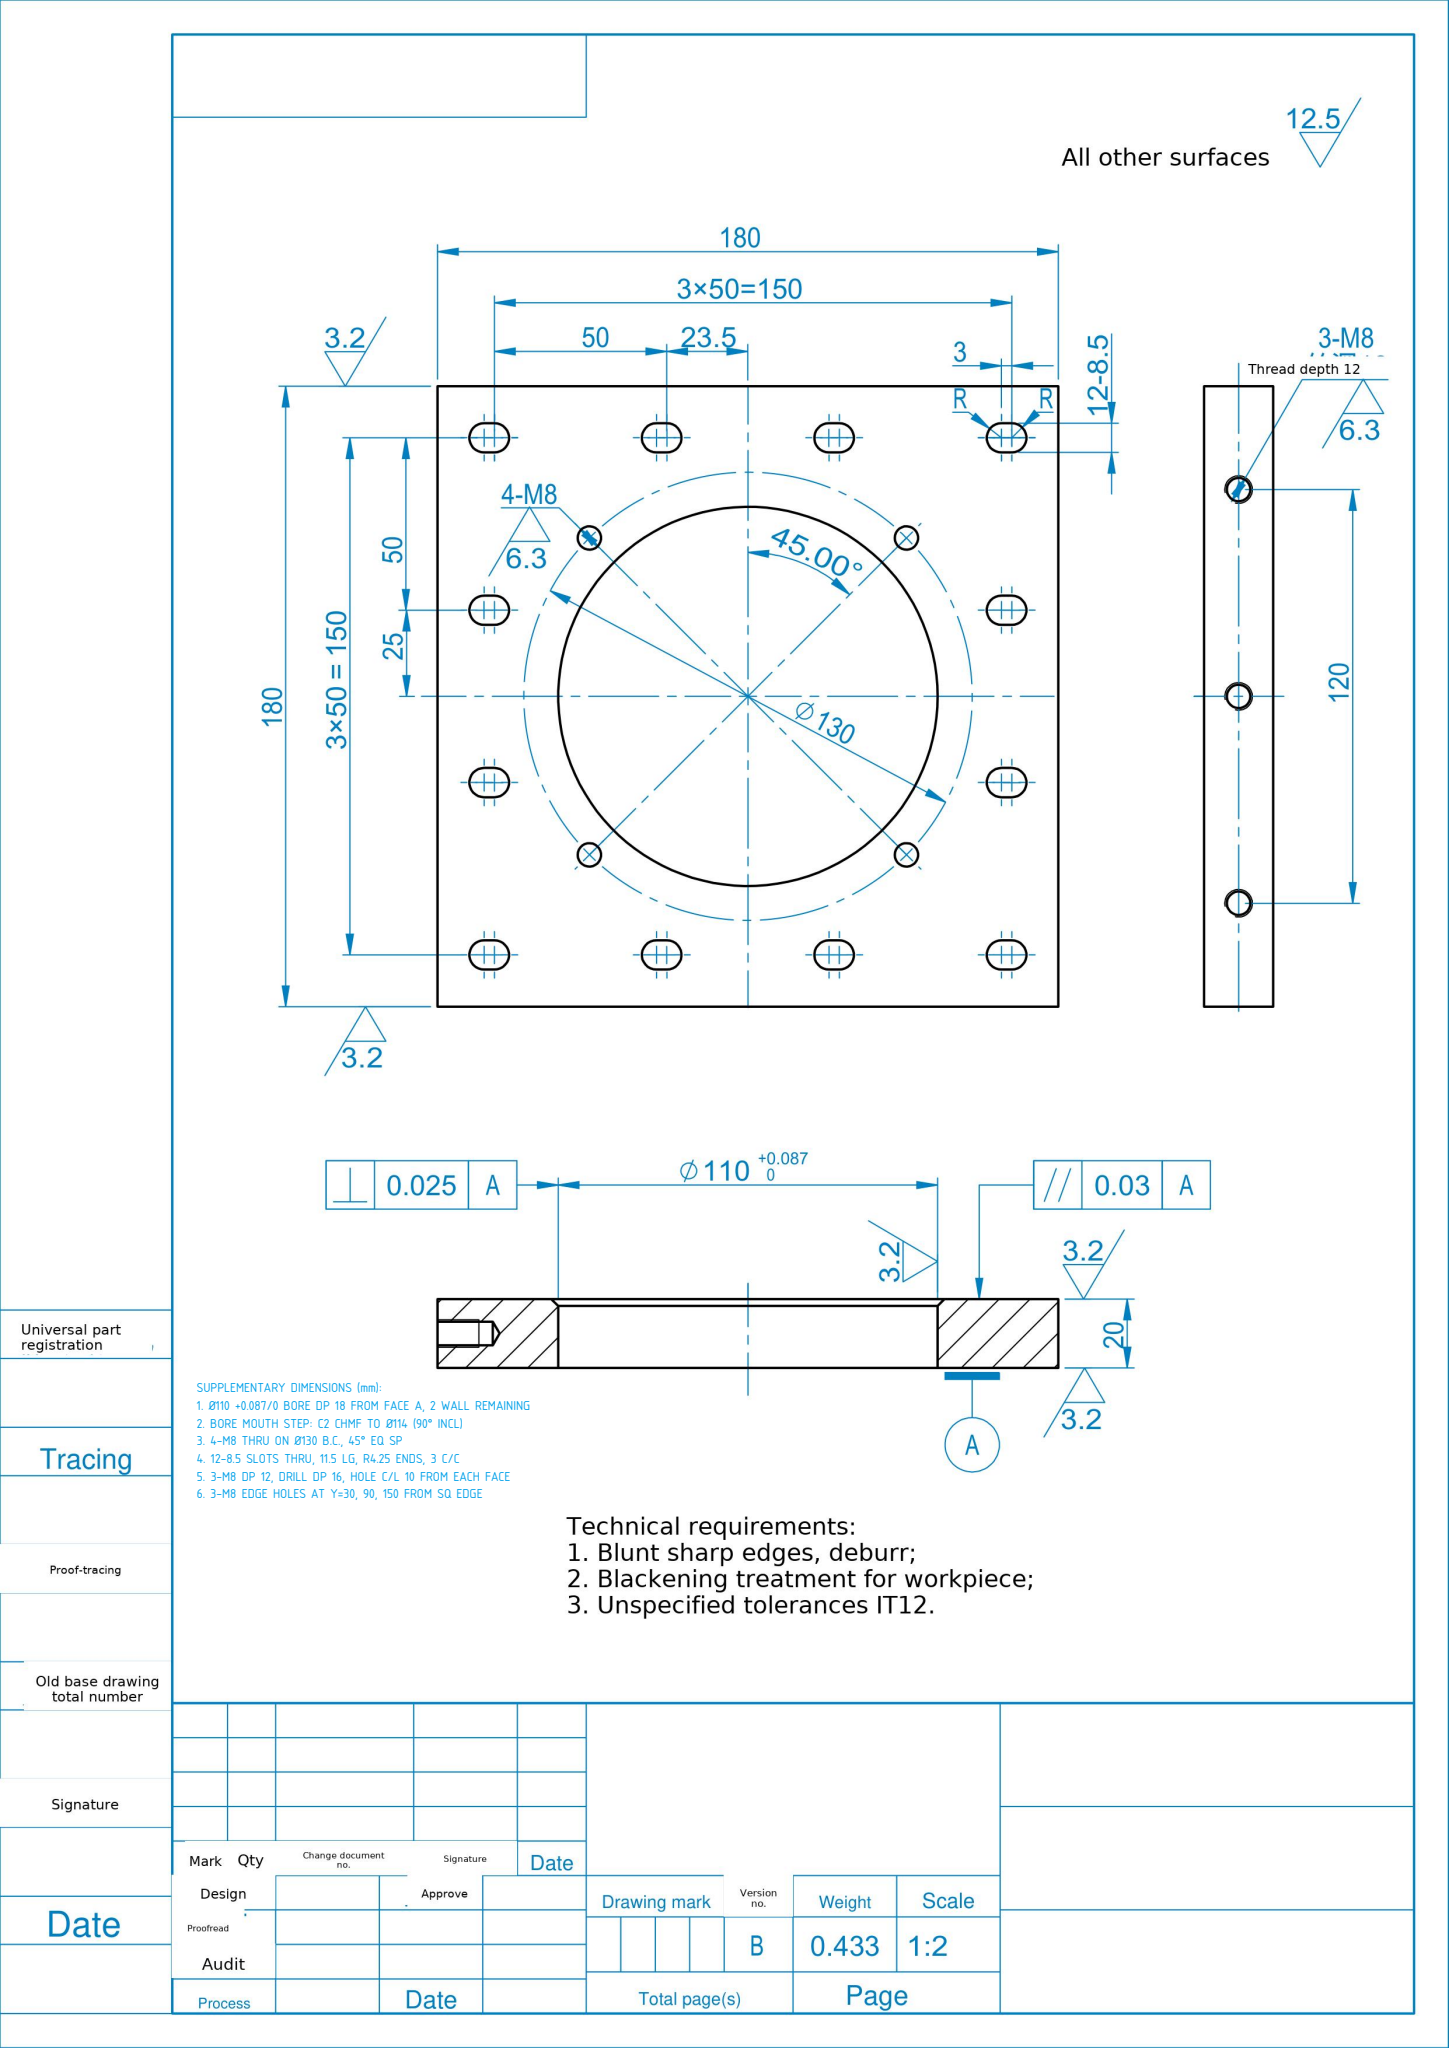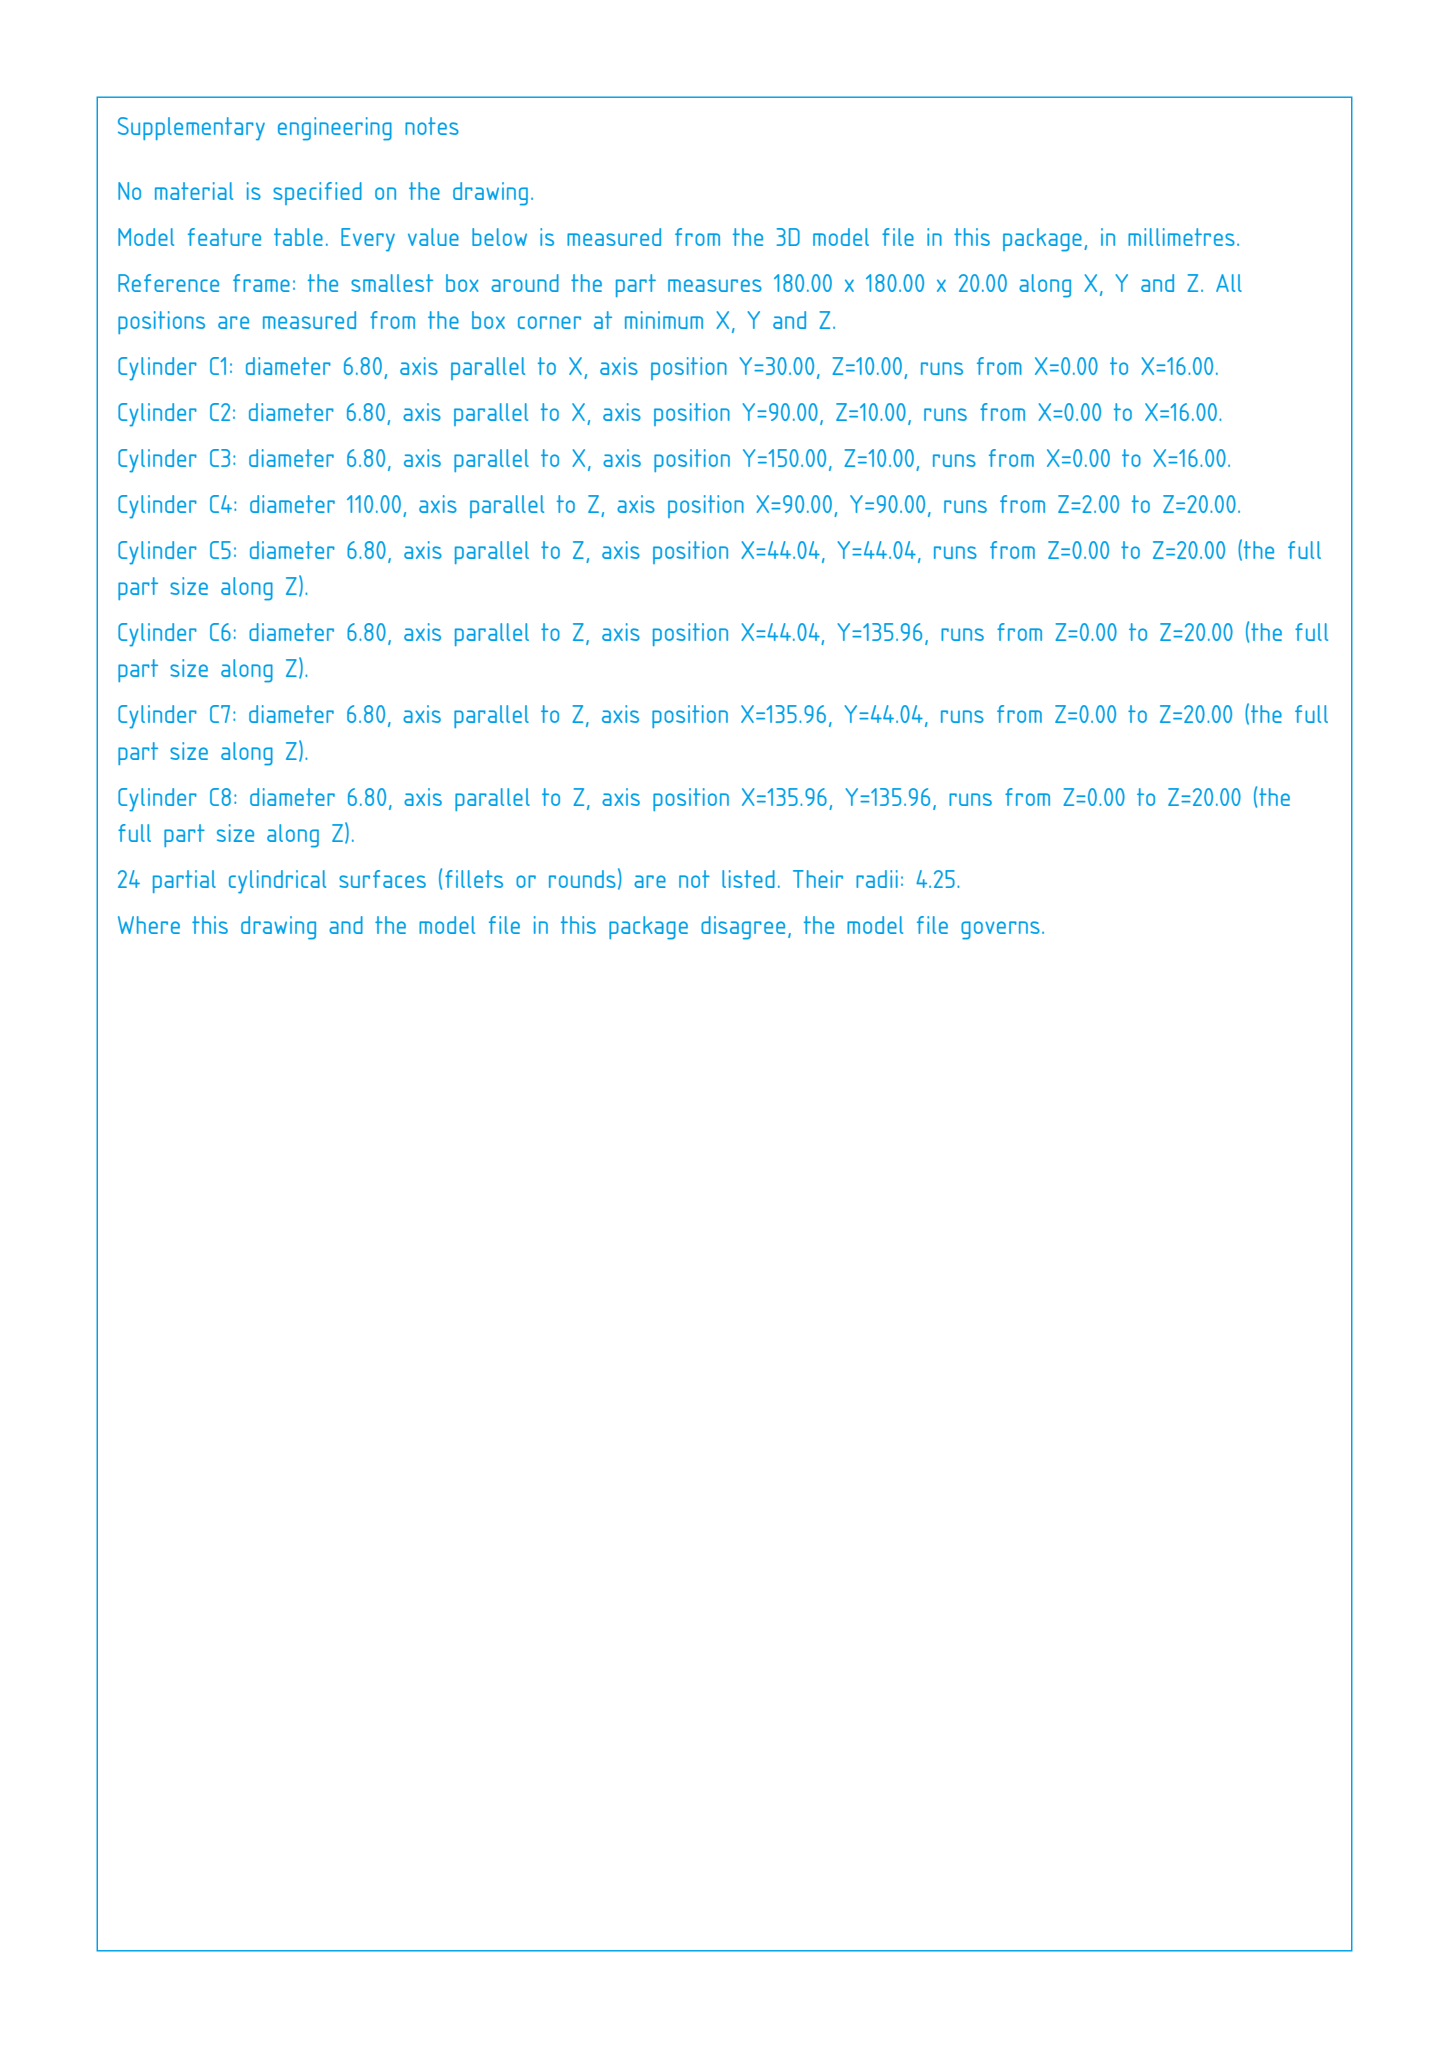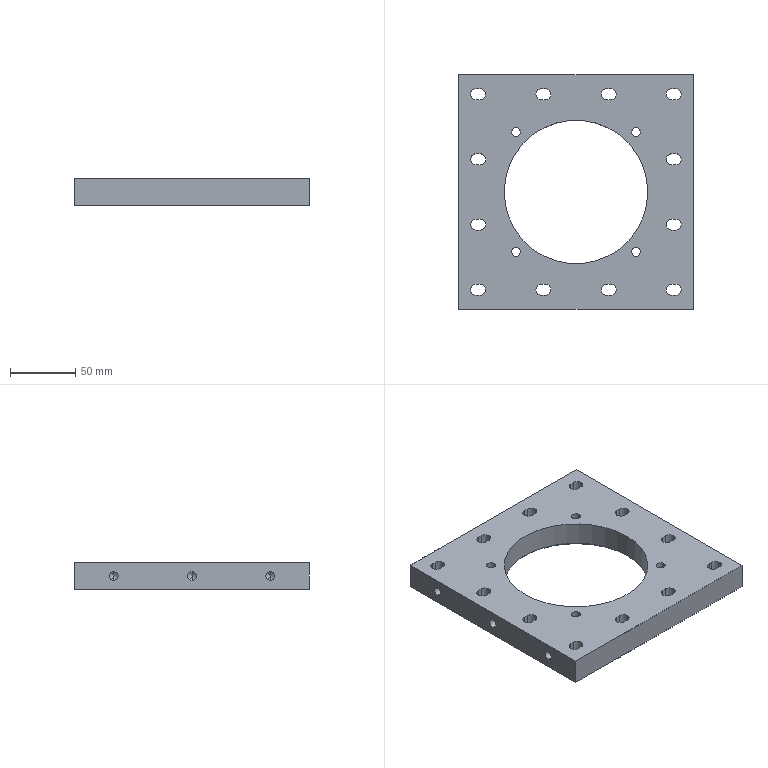Part | SolidWorks | mm | 1 solid | 90 faces | box 180 x 180 x 20 mm | volume 432773 mm3 | cylinder 52 | plane 30 | cone 8 | commonest cylinder face diameters 8.5 x36 6.8 x14 110 x2
build123d program:
from build123d import *

# Parameters (mm, degrees)
SKETCH1_W             = 180
SKETCH1_H             = 180
BOSS_EXTRUDE1_DEPTH   = 10
SKETCH2_R             = 55
CUT_EXTRUDE1_DEPTH    = 129.841
M8_TAPPED_HOLE1_D     = 6.8
CUT_EXTRUDE2_DEPTH    = 129.841
LPATTERN1_COUNT       = 4
LPATTERN1_PITCH       = 50
M8_TAPPED_HOLE3_D     = 6.8
M8_TAPPED_HOLE3_DEPTH = 16
M8_TAPPED_HOLE3_TIP   = 2.043
CHAMFER1_SIZE         = 2


with BuildPart() as part:
    # Sketch1 → Boss-Extrude1 (new, symmetric)
    with BuildSketch(Plane.XY):
        Rectangle(SKETCH1_W, SKETCH1_H)
    extrude(amount=BOSS_EXTRUDE1_DEPTH, both=True)

    # Sketch2 → Cut-Extrude1 (cut, through all)
    with BuildSketch(Plane.XY.offset(10)):
        Circle(SKETCH2_R)
    extrude(amount=-CUT_EXTRUDE1_DEPTH, mode=Mode.SUBTRACT)

    # M8 Tapped Hole1 (through all)
    with Locations(Plane(origin=(0, 0, -10), x_dir=(-1, 0, 0), z_dir=(0, 0, -1))):
        with Locations((45.962, 45.962), (-45.962, 45.962), (-45.962, -45.962), (45.962, -45.962)):
            Hole(M8_TAPPED_HOLE1_D / 2)

    # Sketch6 → Cut-Extrude2 (cut, through all)
    with BuildSketch(Plane(origin=(0, 0, -10), x_dir=(-1, 0, 0), z_dir=(0, 0, -1))):
        with BuildLine():
            Line((73.5, 79.25), (76.5, 79.25))
            ThreePointArc((76.5, 79.25), (80.75, 75), (76.5, 70.75))
            Line((76.5, 70.75), (73.5, 70.75))
            ThreePointArc((73.5, 70.75), (69.25, 75), (73.5, 79.25))
        make_face()
        with BuildLine():
            Line((73.5, -79.25), (76.5, -79.25))
            ThreePointArc((76.5, -79.25), (80.75, -75), (76.5, -70.75))
            Line((76.5, -70.75), (73.5, -70.75))
            ThreePointArc((73.5, -70.75), (69.25, -75), (73.5, -79.25))
        make_face()
        with BuildLine():
            Line((73.5, 29.25), (76.5, 29.25))
            ThreePointArc((76.5, 29.25), (80.75, 25), (76.5, 20.75))
            Line((76.5, 20.75), (73.5, 20.75))
            ThreePointArc((73.5, 20.75), (69.25, 25), (73.5, 29.25))
        make_face()
        with BuildLine():
            Line((73.5, -29.25), (76.5, -29.25))
            ThreePointArc((76.5, -29.25), (80.75, -25), (76.5, -20.75))
            Line((76.5, -20.75), (73.5, -20.75))
            ThreePointArc((73.5, -20.75), (69.25, -25), (73.5, -29.25))
        make_face()
    cut_extrude2 = extrude(amount=-CUT_EXTRUDE2_DEPTH, mode=Mode.SUBTRACT)

    # LPattern1: Cut-Extrude2 ×4
    with Locations(*[(i * LPATTERN1_PITCH, 0, 0) for i in range(1, LPATTERN1_COUNT)]):
        add(cut_extrude2, mode=Mode.SUBTRACT)

    # M8 Tapped Hole3
    with Locations(Plane.ZY.offset(90)):
        with Locations((0, -60), (0, 0), (0, 60)):
            Hole(M8_TAPPED_HOLE3_D / 2, depth=M8_TAPPED_HOLE3_DEPTH)
            with Locations((0, 0, -(M8_TAPPED_HOLE3_DEPTH + M8_TAPPED_HOLE3_TIP / 2))):  # 118° drill point
                Cone(0, M8_TAPPED_HOLE3_D / 2, M8_TAPPED_HOLE3_TIP, mode=Mode.SUBTRACT)

    # Chamfer1
    chamfer1_edges = [part.edges().sort_by_distance(p)[0] for p in [
        (-55, 0, -10),
    ]]
    chamfer(chamfer1_edges, length=CHAMFER1_SIZE)


solid = part.part